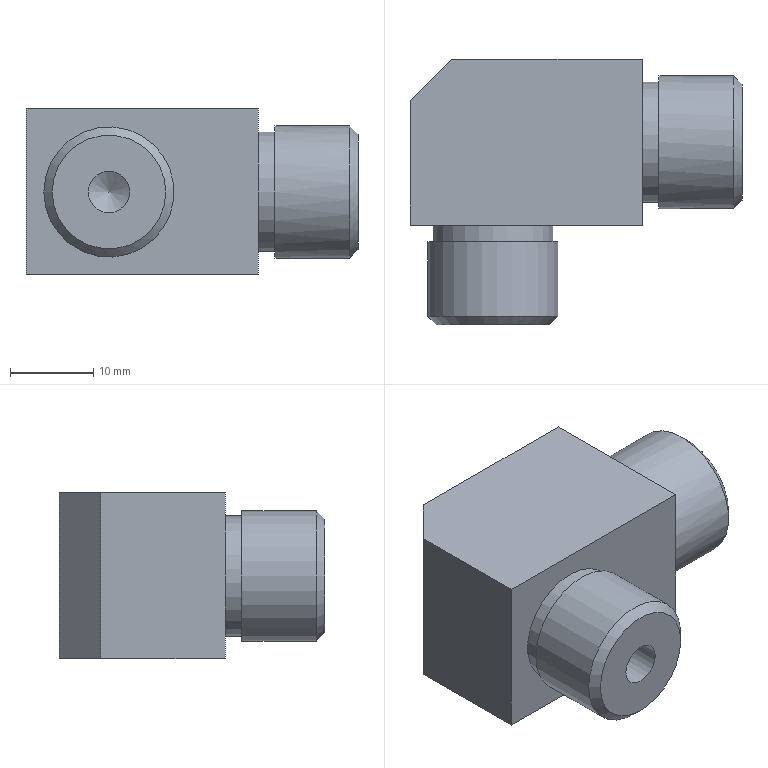Component | NX | CHECK_VALVE_BODY_2 | 1 solid | 26 faces | volume 14233 mm3 | plane 13 | cylinder 8 | cone 5 | commonest cylinder face diameters 14.5 x2 5 x2 16 x1 15.692 x1 8 x1 3 x1